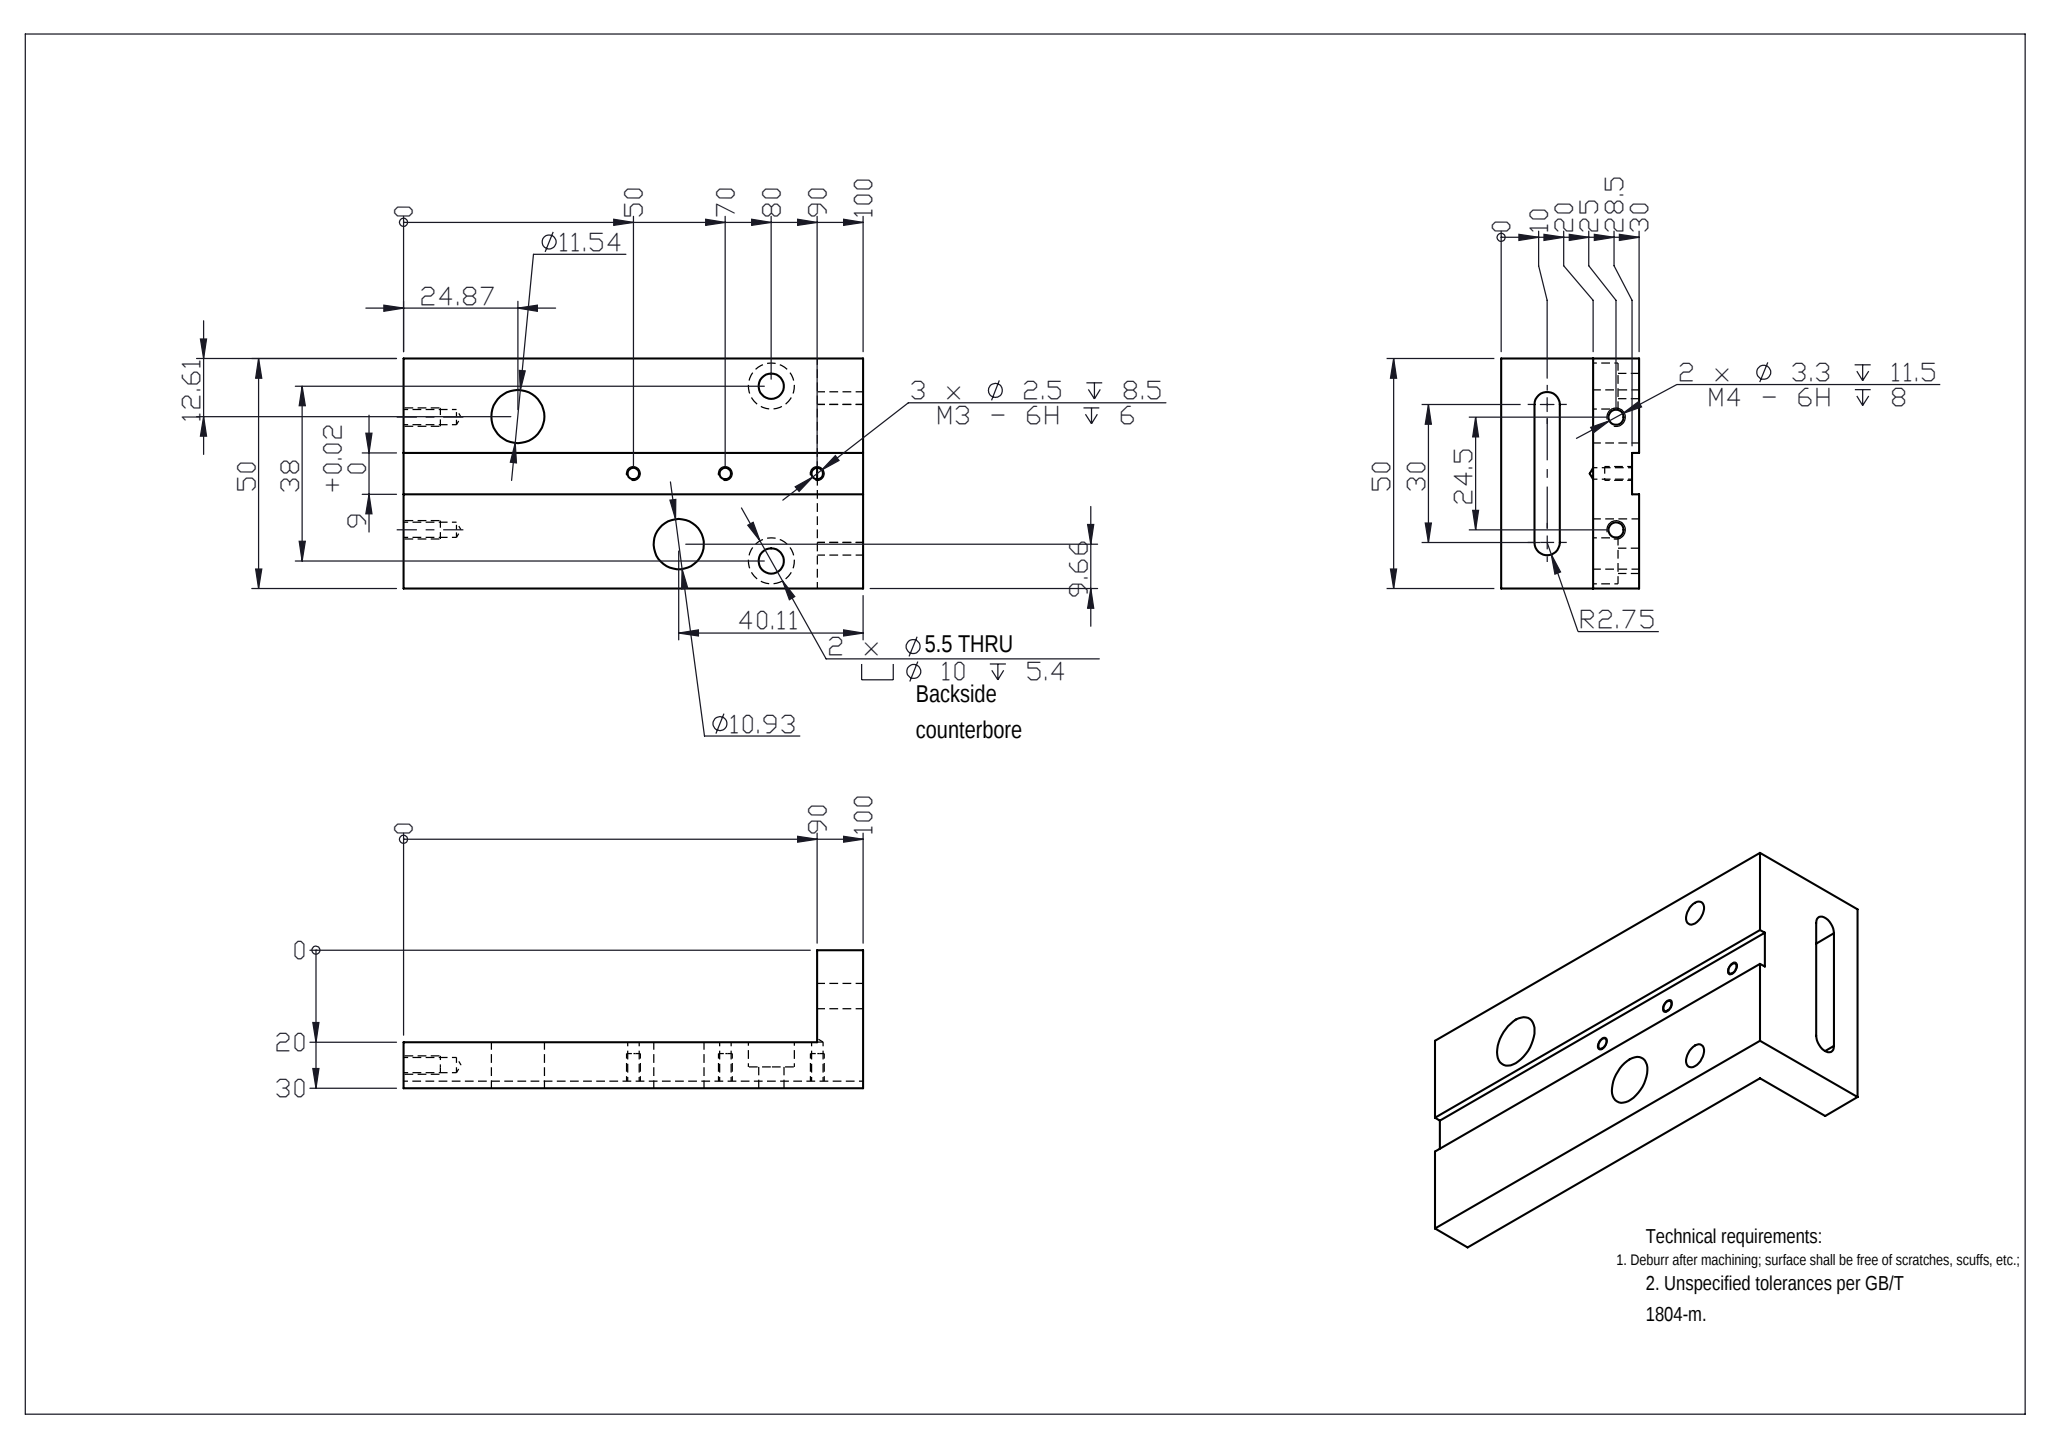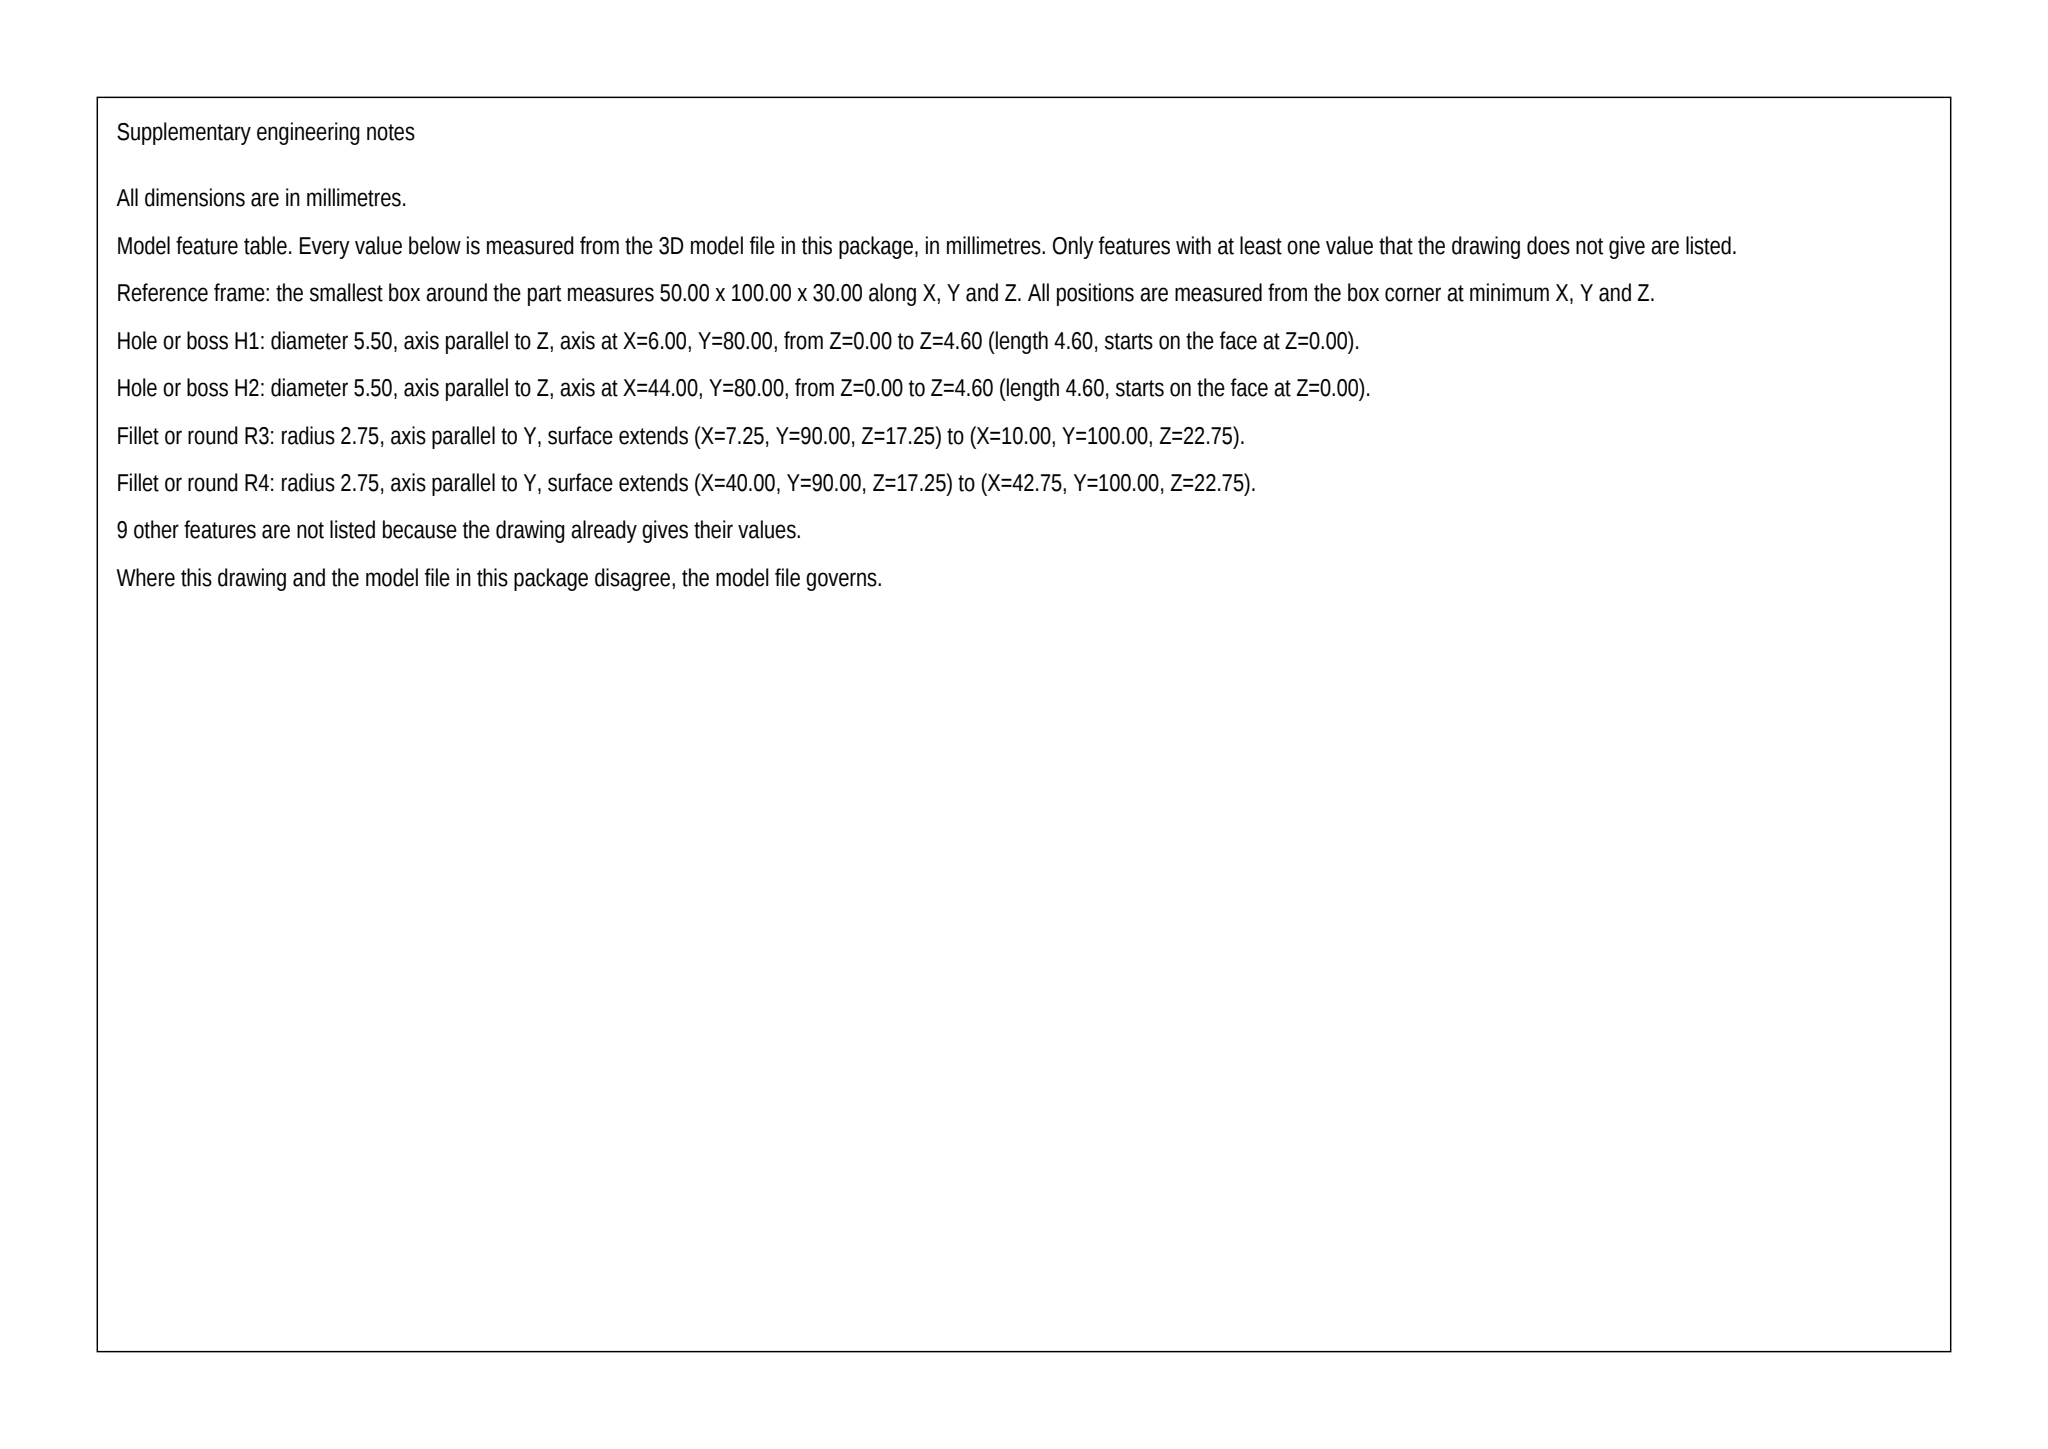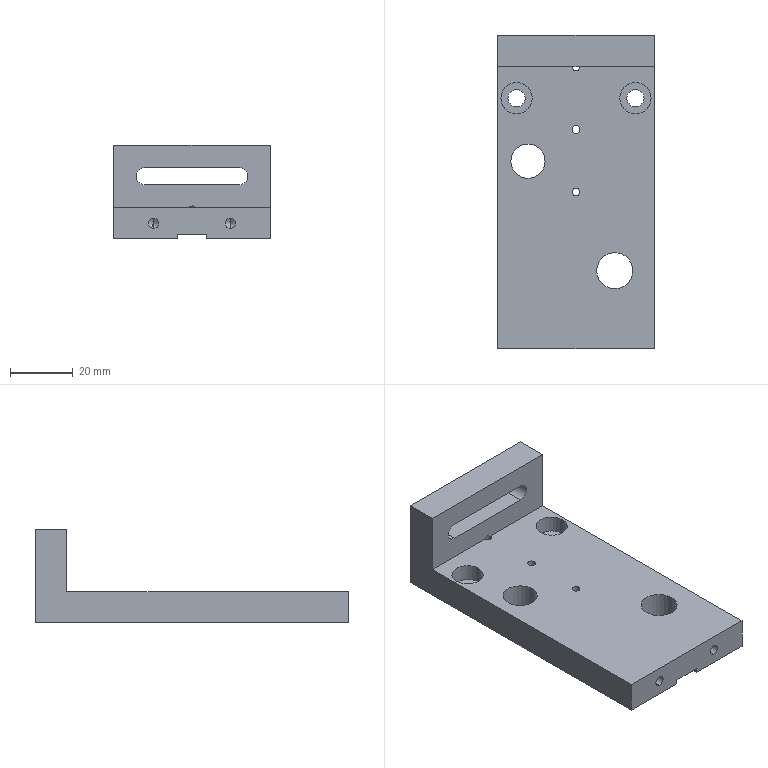Part | SolidWorks | mm | 1 solid | 45 faces | box 50 x 100 x 30 mm | volume 53384 mm3 | cylinder 24 | plane 16 | cone 5 | commonest cylinder face diameters 5.5 x6 2.5 x6 10 x4 3.3 x4 11.541 x2 10.926 x2
Drawing notes:
HORIZ PLATE 10 THK; Ø11.54 & Ø10.93 THRU | from the solid: z=10 plane; Ø11.541 and Ø10.926 z-axis cyls, length 10
GROOVE IN BOT FACE 9 +0.02/0 W x 1.5 DP, CL ON 50 W, FULL 100 LG | from the solid: x-planes 20.5 & 29.5 (9 wide, ctr 25); z=1.5 groove floor, z=0 bottom face split
3 x Ø2.5 / M3-6H ON CL OF 50 W, 25 FROM EACH LONG EDGE | from the solid: Ø2.5 z-cyls at x=25.0, y=50/70/90; bbox x=50 -> mid-width
2 x Ø5.5 THRU, BACKSIDE CBORE Ø10 DP 5.4, 6 FROM EACH LONG EDGE, 38 APART | from the solid: Ø5.5 z-holes at (6,80)&(44,80) L4.6 with coaxial Ø10 bores L5.4 from z=0 face
2 x Ø3.3 / M4-6H CL 5 FROM BOT FACE, 24.5 APART, CTR ON 50 W | from the solid: Ø3.3 y-axis holes at x=12.75 & 37.25, z=5.0; spacing 24.5, ctr x=25
OBROUND SLOT SYMMETRIC ABOUT 50 WIDTH CL; END CTRS 10 FROM EDGES | from the solid: Ø5.5 y-axis cyls at x=10.0 and x=40.0, 30 c-c, midpoint x=25.0 = 50/2
build123d program:
from build123d import *

# Parameters (mm, degrees)
SKETCH1_W                                       = 50
SKETCH1_H                                       = 100
BOSS_EXTRUDE1_DEPTH                             = 10
SKETCH2_W                                       = 50
SKETCH2_H                                       = 10
BOSS_EXTRUDE2_DEPTH                             = 20
SKETCH5_W                                       = 9
SKETCH5_H                                       = 100
CUT_EXTRUDE1_DEPTH                              = 1.5
M3_TAPPED_HOLE1_D                               = 2.5
M3_TAPPED_HOLE1_DEPTH                           = 8.5
M3_TAPPED_HOLE1_TIP                             = 0.7511
M4_TAPPED_HOLE1_D                               = 3.3
M4_TAPPED_HOLE1_DEPTH                           = 11.5
M4_TAPPED_HOLE1_TIP                             = 0.9914
CUT_EXTRUDE2_DEPTH                              = 108.238
M5_HEX_SOCKET_HEAD_CAP_SCREW_CBORE1_D           = 5.5
M5_HEX_SOCKET_HEAD_CAP_SCREW_CBORE1_CBORE_D     = 10
M5_HEX_SOCKET_HEAD_CAP_SCREW_CBORE1_CBORE_DEPTH = 5.4
SKETCH13_R                                      = 5.463
SKETCH13_R_2                                    = 5.771
CUT_EXTRUDE3_DEPTH                              = 10


with BuildPart() as part:
    # Sketch1 → Boss-Extrude1 (new body)
    with BuildSketch(Plane.XY):
        with Locations((25, -50)):
            Rectangle(SKETCH1_W, SKETCH1_H)
    extrude(amount=BOSS_EXTRUDE1_DEPTH)

    # Sketch2 → Boss-Extrude2 (add)
    with BuildSketch(Plane.XY.offset(10)):
        with Locations((25, -5)):
            Rectangle(SKETCH2_W, SKETCH2_H)
    extrude(amount=BOSS_EXTRUDE2_DEPTH)

    # Sketch5 → Cut-Extrude1 (cut)
    with BuildSketch(Plane(origin=(0, 0, 0), x_dir=(-1, 0, 0), z_dir=(0, 0, -1))):
        with Locations((-25, -50)):
            Rectangle(SKETCH5_W, SKETCH5_H)
    extrude(amount=-CUT_EXTRUDE1_DEPTH, mode=Mode.SUBTRACT)

    # M3 Tapped Hole1
    with Locations(Plane(origin=(0, 0, 1.5), x_dir=(-1, 0, 0), z_dir=(0, 0, -1))):
        with Locations((-25, -10), (-25, -30), (-25, -50)):
            Hole(M3_TAPPED_HOLE1_D / 2, depth=M3_TAPPED_HOLE1_DEPTH)
            with Locations((0, 0, -(M3_TAPPED_HOLE1_DEPTH + M3_TAPPED_HOLE1_TIP / 2))):  # 118° drill point
                Cone(0, M3_TAPPED_HOLE1_D / 2, M3_TAPPED_HOLE1_TIP, mode=Mode.SUBTRACT)

    # M4 Tapped Hole1
    with Locations(Plane(origin=(0, -100, 0), x_dir=(-1, 0, 0), z_dir=(0, -1, 0))):
        with Locations((-37.25, -5), (-12.75, -5)):
            Hole(M4_TAPPED_HOLE1_D / 2, depth=M4_TAPPED_HOLE1_DEPTH)
            with Locations((0, 0, -(M4_TAPPED_HOLE1_DEPTH + M4_TAPPED_HOLE1_TIP / 2))):  # 118° drill point
                Cone(0, M4_TAPPED_HOLE1_D / 2, M4_TAPPED_HOLE1_TIP, mode=Mode.SUBTRACT)

    # Sketch10 → Cut-Extrude2 (cut, through all)
    with BuildSketch(Plane.XZ.offset(10)):
        with BuildLine():
            Line((40, 17.25), (10, 17.25))
            ThreePointArc((10, 17.25), (7.25, 20), (10, 22.75))
            Line((10, 22.75), (40, 22.75))
            ThreePointArc((40, 22.75), (42.75, 20), (40, 17.25))
        make_face()
    extrude(amount=-CUT_EXTRUDE2_DEPTH, mode=Mode.SUBTRACT)

    # M5 Hex Socket Head Cap Screw CBORE1 (through all)
    with Locations(Plane.XY.offset(10)):
        with Locations((44, -20), (6, -20)):
            CounterBoreHole(M5_HEX_SOCKET_HEAD_CAP_SCREW_CBORE1_D / 2, M5_HEX_SOCKET_HEAD_CAP_SCREW_CBORE1_CBORE_D / 2, M5_HEX_SOCKET_HEAD_CAP_SCREW_CBORE1_CBORE_DEPTH)

    # Sketch13 → Cut-Extrude3 (cut)
    with BuildSketch(Plane.XY.offset(10)):
        with Locations((9.656, -40.115)):
            Circle(SKETCH13_R)
        with Locations((37.393, -75.131)):
            Circle(SKETCH13_R_2)
    extrude(amount=-CUT_EXTRUDE3_DEPTH, mode=Mode.SUBTRACT)


solid = part.part